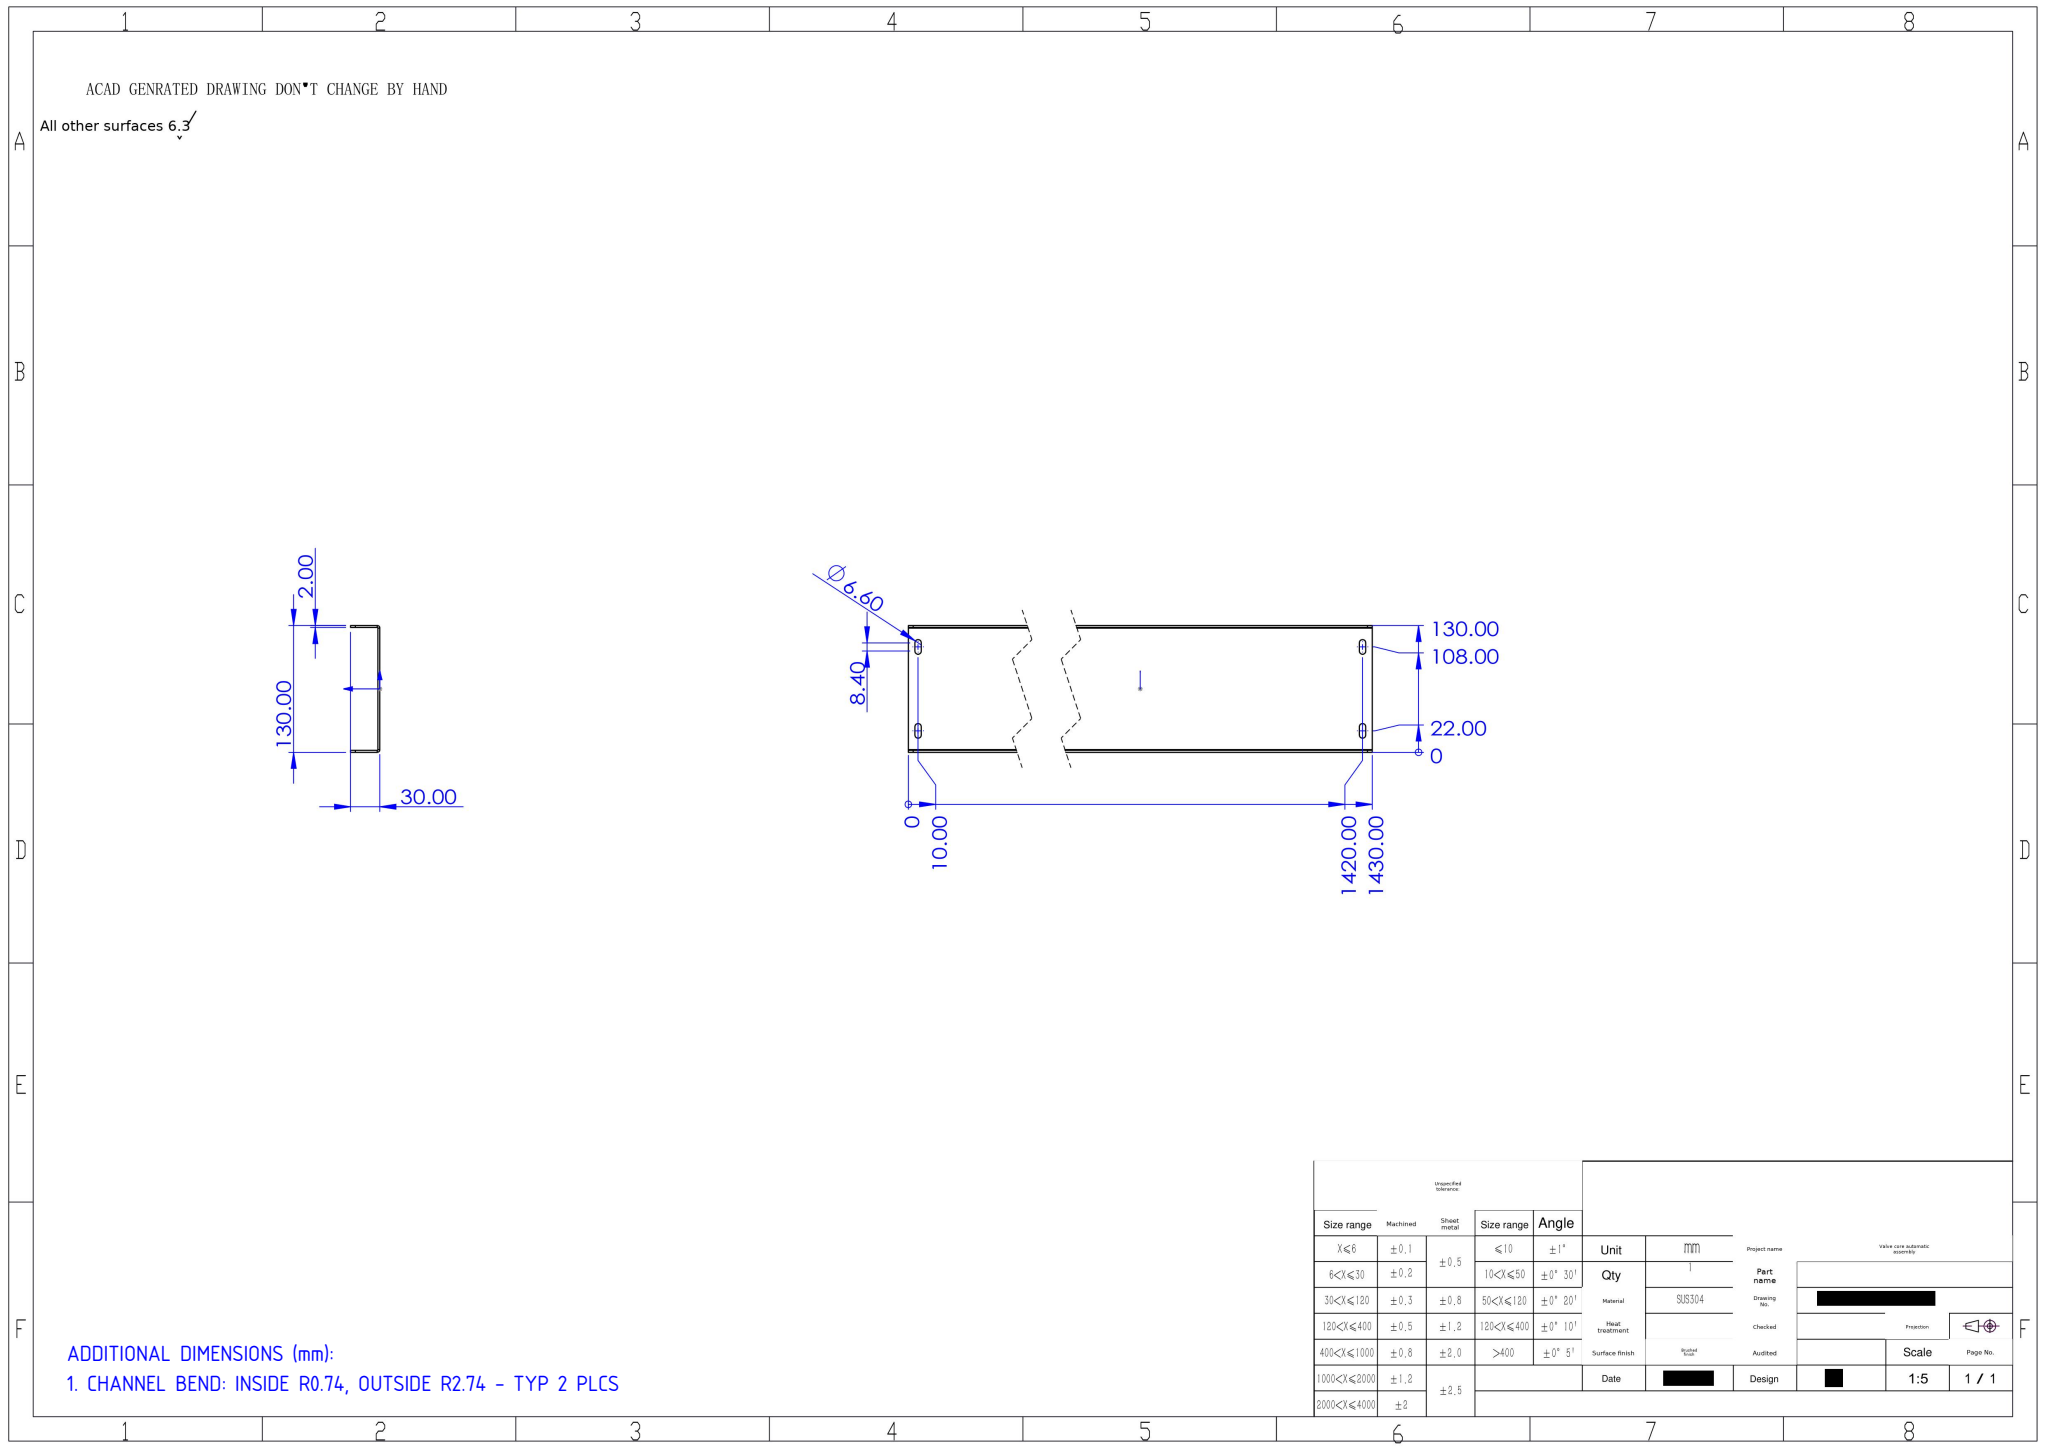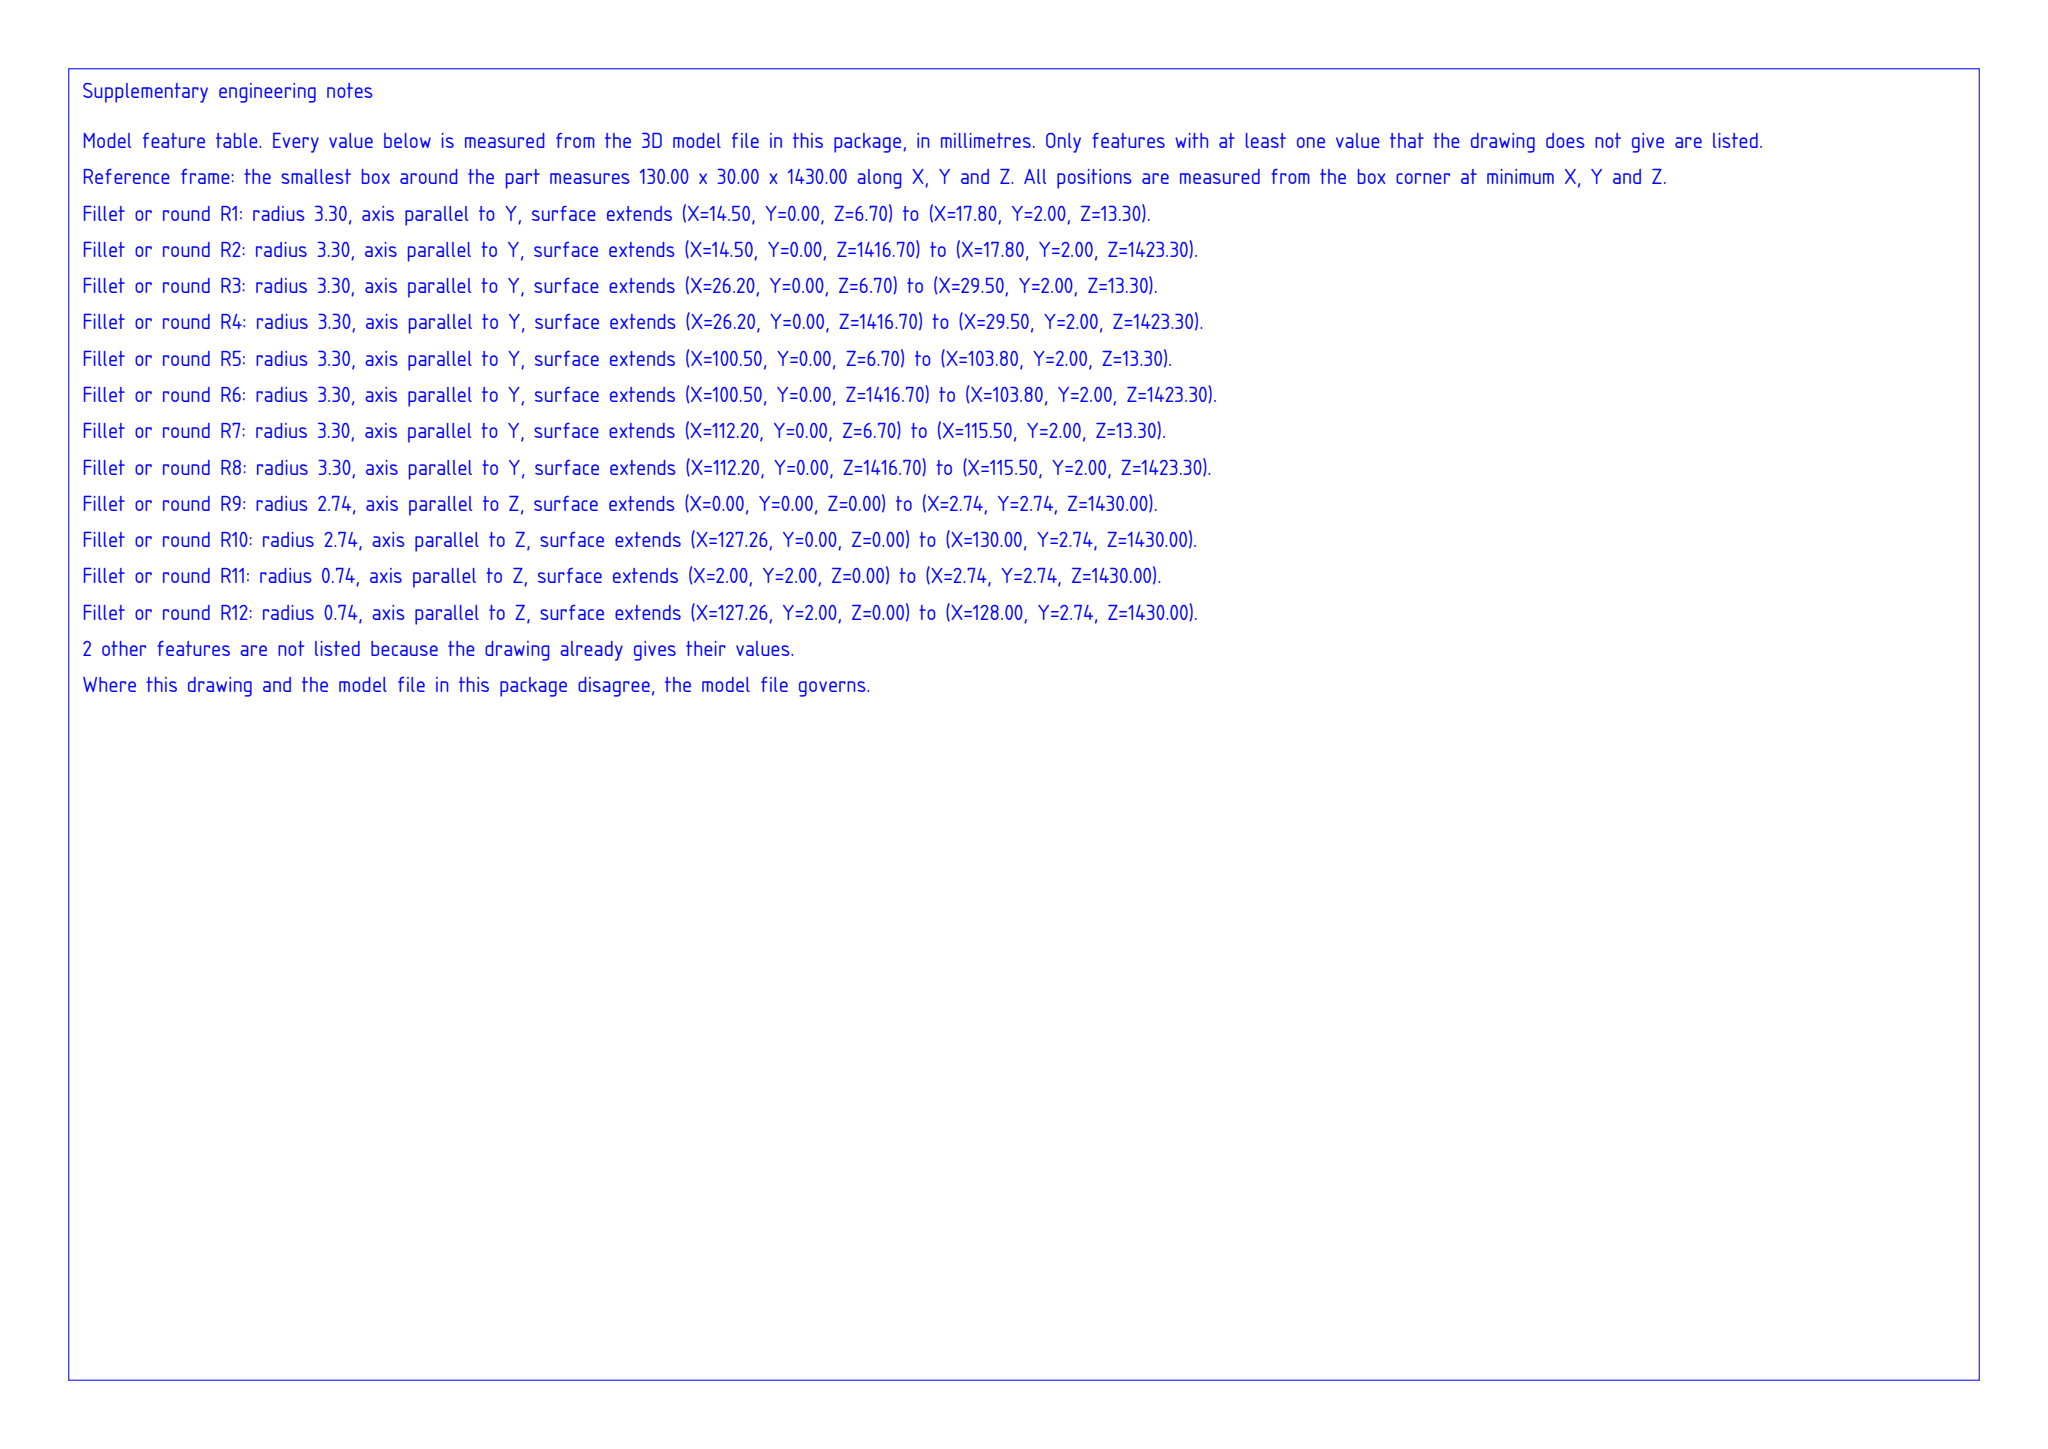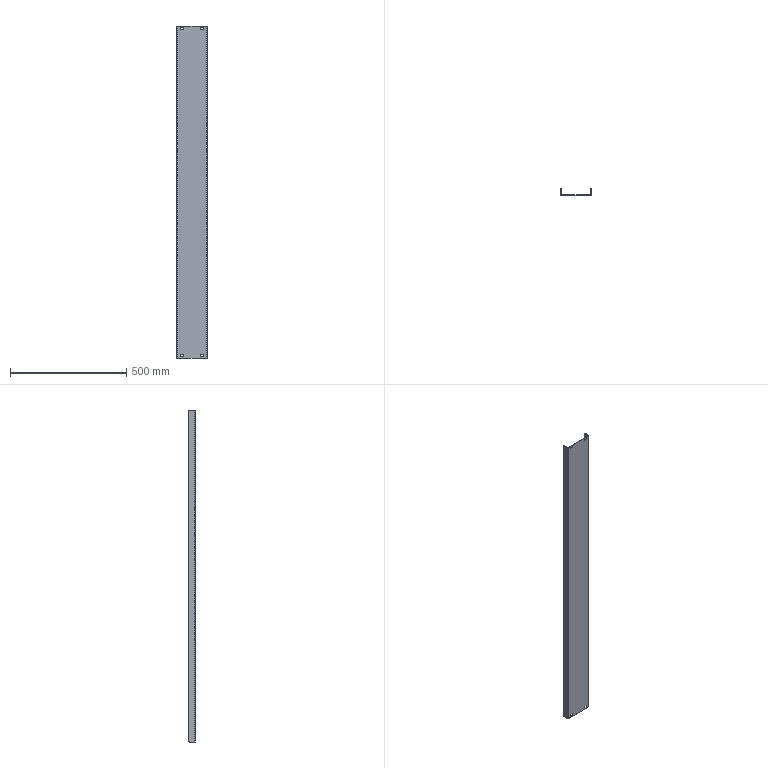Part | SolidWorks | mm | 1 solid | 42 faces | box 130 x 30 x 1430 mm | volume 526936 mm3 | plane 26 | cylinder 16 | commonest cylinder face diameters 6.6 x8 10 x4 1.473 x2 5.473 x2